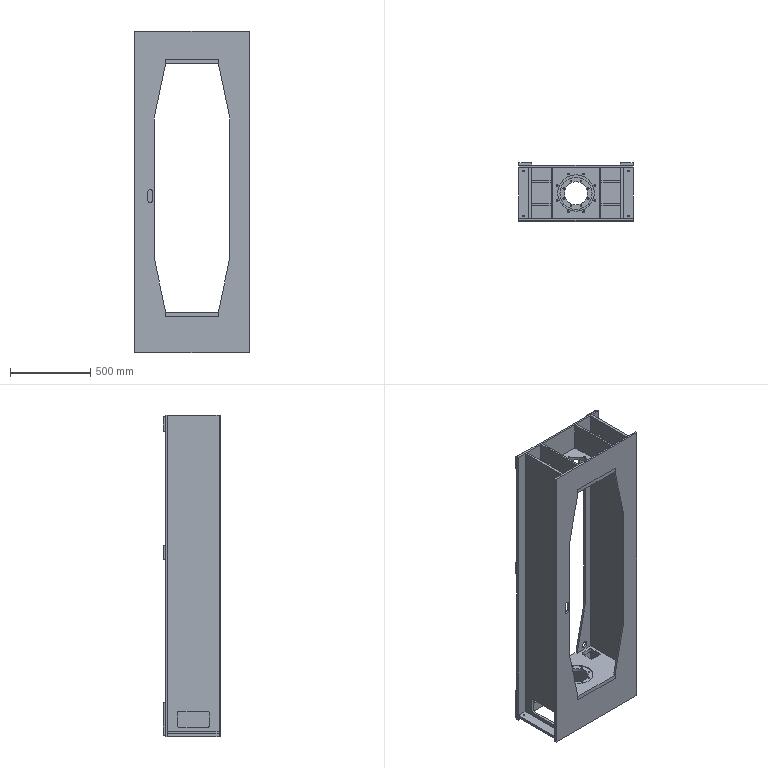Assembly | NX | mm | 24 component files | 24 solids | 322 faces | box 710 x 360 x 2000 mm | volume 50695894 mm3 | plane 212 | cylinder 66 | cone 44 | commonest cylinder face diameters 20 x24 11.5 x18 9.5 x12 40 x6 30 x2 144 x1 200 x1 226 x1
Bill of materials:
CH3404.5-8 | 1 |  | Plain solid rectangular plate (thin cuboid) with no visible holes or cutouts.
CH3404.5-12 | 1 |  | Plain solid rectangular plate (thin cuboid) with no visible holes or cutouts.
CH3404.5-13 | 2 |  | Thick rectangular bar/plate with three equally spaced round through-holes on its long centerline.
CH3404.5-14 | 4 |  | Thick, roughly square plate with one centered round through-hole.
CH3404.5-5 | 1 |  | Flat plate with a large central circular opening surrounded by eight small holes evenly spaced on a circle. The outline has stepped tabs: the middle section sticks out past the end sections along both long edges.
CH3404.5-10 | 2 |  | Long rectangular flat bar with one round through-hole near each end.
CH3404.5-1 | 1 |  | Thin, long rectangular sheet strip with one small rounded-rectangle slot near one end.
CH3404.5-4 | 2 |  | Plain solid rectangular block/bar, longer than it is tall, with no visible features.
CH3404.5-2 | 1 |  | Thin rectangular sheet frame with a large elongated octagonal-style cutout (chamfered/tapered ends) and one small vertical slot on one side.
CH3404.5-11 | 1 |  | Thin, long rectangular sheet strip with one small rounded-rectangle slot near one end.
CH3404.5-7 | 1 |  | Thin rectangular sheet frame with a large elongated cutout with tapered ends, six small round holes in the border, and two small rounded-square cutouts near one end.
CH3404.5-3 | 2 |  | Plain solid rectangular plate with no visible holes or cutouts.
CH3404.5-9 | 4 |  | Plain rectangular solid block (thick flat plate); rectangular main face, roughly 1.8:1 aspect, with sharp edges and no visible holes, cutouts, chamfers or other features.
CH3404.5-6 | 1 |  | Flat plate of uniform thickness with a stepped outline: a center section wider than the two end sections, forming shallow shoulders on both long edges. It has a large central circular through-hole surrounded by a shallow annular recess or counterbore, eight small through-holes evenly spaced on a circle around the central hole, and two rounded-rectangle through-cutouts, one near each end.
Mates:
1. fix | CH3404_5-6 1 component
2. touch align | CH3404_5-3 2 face | CH3404_5-6 1 face
3. touch align | CH3404_5-3 2 face | CH3404_5-6 1 face
4. distance | CH3404_5-3 2 face | assembly datumplane
5. touch align | CH3404_5-3 1 face | CH3404_5-6 1 face
6. touch align | CH3404_5-3 1 face | CH3404_5-6 1 face
7. distance | CH3404_5-3 1 face | assembly datumplane
8. touch align | CH3404_5-4 2 face | CH3404_5-6 1 face
9. touch align | CH3404_5-4 2 face | CH3404_5-6 1 face
10. touch align | CH3404_5-4 1 face | CH3404_5-6 1 face
11. touch align | CH3404_5-2 1 face | CH3404_5-6 1 face
12. touch align | CH3404_5-2 1 face | CH3404_5-3 1 face
13. touch align | CH3404_5-2 1 face | CH3404_5-6 1 face
14. touch align | CH3404_5-7 1 face | CH3404_5-6 1 face
15. touch align | CH3404_5-7 1 face | CH3404_5-3 1 face
16. touch align | CH3404_5-1 1 face | CH3404_5-6 1 face
17. touch align | CH3404_5-1 1 face | CH3404_5-3 1 face
18. touch align | CH3404_5-1 1 face | CH3404_5-2 1 face
19. touch align | CH3404_5-5 1 face | CH3404_5-2 1 face
20. touch align | CH3404_5-5 1 face | CH3404_5-7 1 face
21. touch align | CH3404_5-5 1 face | CH3404_5-6 1 face
22. touch align | CH3404_5-8 1 face | CH3404_5-5 1 face
23. touch align | CH3404_5-8 1 face | CH3404_5-6 1 face
24. distance | CH3404_5-8 1 face | assembly datumplane
25. touch align | CH3404_5-9 4 face | CH3404_5-6 1 face
26. touch align | CH3404_5-9 4 face | CH3404_5-5 1 face
27. distance | CH3404_5-9 4 face | assembly datumplane
28. touch align | CH3404_5-9 3 face | CH3404_5-6 1 face
29. touch align | CH3404_5-9 3 face | CH3404_5-5 1 face
30. distance | CH3404_5-9 3 face | assembly datumplane
31. touch align | CH3404_5-9 2 face | CH3404_5-6 1 face
32. touch align | CH3404_5-9 2 face | CH3404_5-5 1 face
33. distance | CH3404_5-9 2 face | assembly datumplane
34. touch align | CH3404_5-9 1 face | CH3404_5-6 1 face
35. touch align | CH3404_5-9 1 face | CH3404_5-5 1 face
36. distance | CH3404_5-9 1 face | assembly datumplane
37. touch align | CH3404_5-11 1 face | CH3404_5-6 1 face
38. touch align | CH3404_5-11 1 face | CH3404_5-3 1 face
39. touch align | CH3404_5-12 1 face | CH3404_5-2 1 face
40. touch align | CH3404_5-12 1 face | CH3404_5-5 1 face
41. touch align | CH3404_5-12 1 face | CH3404_5-9 4 face
42. touch align | CH3404_5-13 2 face | CH3404_5-7 1 face
43. touch align | CH3404_5-13 2 face | CH3404_5-7 1 face
44. distance | CH3404_5-13 2 face | CH3404_5-7 1 face
45. touch align | CH3404_5-13 1 face | CH3404_5-7 1 face
46. touch align | CH3404_5-13 1 face | CH3404_5-7 1 face
47. touch align | CH3404_5-13 1 face | CH3404_5-13 2 face
48. touch align | CH3404_5-7 1 face | CH3404_5-6 1 face
49. touch align | CH3404_5-10 2 face | CH3404_5-7 1 face
50. distance | CH3404_5-10 2 face | CH3404_5-2 1 face
51. touch align | CH3404_5-10 1 face | CH3404_5-2 1 face
52. distance | CH3404_5-10 1 face | CH3404_5-7 1 face
53. touch align | CH3404_5-10 2 face | CH3404_5-2 1 face
54. touch align | CH3404_5-10 1 face | CH3404_5-7 1 face
55. touch align | CH3404_5-4 1 | assembly datumplane
56. touch align | CH3404_5-4 2 face | CH3404_5-4 1 face
57. touch align | CH3404_5-14 4 face | CH3404_5-7 1 face
58. touch align | CH3404_5-14 4 face | CH3404_5-7 1 face
59. distance | CH3404_5-14 4 face | CH3404_5-7 1 face
60. touch align | CH3404_5-14 3 face | CH3404_5-7 1 face
61. touch align | CH3404_5-14 3 face | CH3404_5-7 1 face
62. touch align | CH3404_5-14 3 face | CH3404_5-14 4 face
63. touch align | CH3404_5-14 2 face | CH3404_5-7 1 face
64. touch align | CH3404_5-14 2 face | CH3404_5-7 1 face
65. distance | CH3404_5-14 2 face | CH3404_5-7 1 face
66. touch align | CH3404_5-14 1 face | CH3404_5-7 1 face
67. touch align | CH3404_5-14 1 face | CH3404_5-7 1 face
68. touch align | CH3404_5-14 1 face | CH3404_5-14 2 face